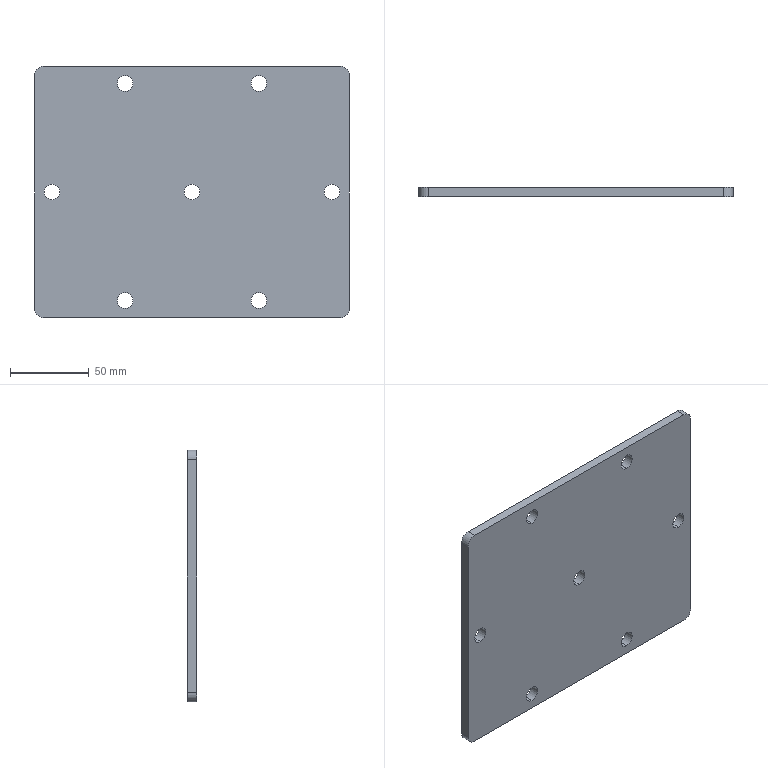Component | SolidWorks | UpperHousingAssembly-1_PeepHoleCover-1 | 1 solid | 24 faces | box 200 x 6 x 160 mm | volume 188516 mm3 | cylinder 18 | plane 6 | commonest cylinder face diameters 10 x14 12 x4
build123d program:
from build123d import *

# Parameters (mm, degrees)
SKETCH1_W           = 200
SKETCH1_H           = 160
BOSS_EXTRUDE1_DEPTH = 6
FILLET1_R           = 6
M10_TAPPED_HOLE1_D  = 10


with BuildPart() as part:
    # Sketch1 → Boss-Extrude1 (new body)
    with BuildSketch(Plane(origin=(0, 0, 0), x_dir=(1, 0, 0), z_dir=(0, 1, 0))):
        Rectangle(SKETCH1_W, SKETCH1_H)
    extrude(amount=BOSS_EXTRUDE1_DEPTH)

    # Fillet1
    fillet1_edges = [part.edges().sort_by_distance(p)[0] for p in [
        (100, 3, 80),
        (-100, 3, 80),
        (-100, 3, -80),
        (100, 3, -80),
    ]]
    fillet(fillet1_edges, radius=FILLET1_R)

    # M10 Tapped Hole1 (through all)
    with Locations(Plane(origin=(0, 6, 0), x_dir=(1, 0, 0), z_dir=(0, 1, 0))):
        with Locations((0, 0), (42.5, 69), (-42.5, 69), (-89, 0), (89, 0), (42.5, -69), (-42.5, -69)):
            Hole(M10_TAPPED_HOLE1_D / 2)


solid = part.part

# Placed as in the assembly
solid = solid.moved(Location((895.83, 1541.591, 1632.217), (0, 0, 0)))
STEP:
#1=COLOUR_RGB('',0.7922,0.8196,0.9333);
#2=FILL_AREA_STYLE_COLOUR('',#1);
#3=FILL_AREA_STYLE('',(#2));
#4=SURFACE_STYLE_FILL_AREA(#3);
#5=SURFACE_SIDE_STYLE('',(#4));
#6=SURFACE_STYLE_USAGE(.BOTH.,#5);
#7=PRESENTATION_STYLE_ASSIGNMENT((#6));
#8=CARTESIAN_POINT('',(35.269,60.693,64.064));
#9=VERTEX_POINT('',#8);
#10=CARTESIAN_POINT('',(35.269,60.693,64.457));
#11=VERTEX_POINT('',#10);
#12=CARTESIAN_POINT('',(35.269,60.693,64.26));
#13=DIRECTION('',(0.,1.,0.));
#14=DIRECTION('',(0.,0.,1.));
#15=AXIS2_PLACEMENT_3D('',#12,#13,#14);
#16=CIRCLE('',#15,0.1969);
#17=EDGE_CURVE('',#9,#11,#16,.T.);
#18=ORIENTED_EDGE('',*,*,#17,.F.);
#19=CARTESIAN_POINT('',(35.269,60.929,64.064));
#20=VERTEX_POINT('',#19);
#21=CARTESIAN_POINT('',(35.269,60.929,64.064));
#22=DIRECTION('',(0.,1.,0.));
#23=VECTOR('',#22,39.37);
#24=LINE('',#21,#23);
#25=EDGE_CURVE('',#9,#20,#24,.T.);
#26=ORIENTED_EDGE('',*,*,#25,.T.);
#27=CARTESIAN_POINT('',(35.269,60.929,64.457));
#28=VERTEX_POINT('',#27);
#29=CARTESIAN_POINT('',(35.269,60.929,64.26));
#30=DIRECTION('',(0.,1.,0.));
#31=DIRECTION('',(0.,0.,1.));
#32=AXIS2_PLACEMENT_3D('',#29,#30,#31);
#33=CIRCLE('',#32,0.1969);
#34=EDGE_CURVE('',#20,#28,#33,.T.);
#35=ORIENTED_EDGE('',*,*,#34,.T.);
#36=CARTESIAN_POINT('',(35.269,60.929,64.457));
#37=DIRECTION('',(0.,1.,0.));
#38=VECTOR('',#37,39.37);
#39=LINE('',#36,#38);
#40=EDGE_CURVE('',#11,#28,#39,.T.);
#41=ORIENTED_EDGE('',*,*,#40,.F.);
#42=EDGE_LOOP('',(#18,#26,#35,#41));
#43=FACE_OUTER_BOUND('',#42,.T.);
#44=CARTESIAN_POINT('',(35.269,60.929,64.26));
#45=DIRECTION('',(0.,1.,0.));
#46=DIRECTION('',(0.,0.,1.));
#47=AXIS2_PLACEMENT_3D('',#44,#45,#46);
#48=CYLINDRICAL_SURFACE('',#47,0.1969);
#49=ADVANCED_FACE('',(#43),#48,.F.);
#50=CARTESIAN_POINT('',(36.942,60.693,61.347));
#51=VERTEX_POINT('',#50);
#52=CARTESIAN_POINT('',(36.942,60.693,61.741));
#53=VERTEX_POINT('',#52);
#54=CARTESIAN_POINT('',(36.942,60.693,61.544));
#55=DIRECTION('',(0.,1.,0.));
#56=DIRECTION('',(0.,0.,1.));
#57=AXIS2_PLACEMENT_3D('',#54,#55,#56);
#58=CIRCLE('',#57,0.1969);
#59=EDGE_CURVE('',#51,#53,#58,.T.);
#60=ORIENTED_EDGE('',*,*,#59,.F.);
#61=CARTESIAN_POINT('',(36.942,60.929,61.347));
#62=VERTEX_POINT('',#61);
#63=CARTESIAN_POINT('',(36.942,60.929,61.347));
#64=DIRECTION('',(0.,1.,0.));
#65=VECTOR('',#64,39.37);
#66=LINE('',#63,#65);
#67=EDGE_CURVE('',#51,#62,#66,.T.);
#68=ORIENTED_EDGE('',*,*,#67,.T.);
#69=CARTESIAN_POINT('',(36.942,60.929,61.741));
#70=VERTEX_POINT('',#69);
#71=CARTESIAN_POINT('',(36.942,60.929,61.544));
#72=DIRECTION('',(0.,1.,0.));
#73=DIRECTION('',(0.,0.,1.));
#74=AXIS2_PLACEMENT_3D('',#71,#72,#73);
#75=CIRCLE('',#74,0.1969);
#76=EDGE_CURVE('',#62,#70,#75,.T.);
#77=ORIENTED_EDGE('',*,*,#76,.T.);
#78=CARTESIAN_POINT('',(36.942,60.929,61.741));
#79=DIRECTION('',(0.,1.,0.));
#80=VECTOR('',#79,39.37);
#81=LINE('',#78,#80);
#82=EDGE_CURVE('',#53,#70,#81,.T.);
#83=ORIENTED_EDGE('',*,*,#82,.F.);
#84=EDGE_LOOP('',(#60,#68,#77,#83));
#85=FACE_OUTER_BOUND('',#84,.T.);
#86=CARTESIAN_POINT('',(36.942,60.929,61.544));
#87=DIRECTION('',(0.,1.,0.));
#88=DIRECTION('',(0.,0.,1.));
#89=AXIS2_PLACEMENT_3D('',#86,#87,#88);
#90=CYLINDRICAL_SURFACE('',#89,0.1969);
#91=ADVANCED_FACE('',(#85),#90,.F.);
#92=CARTESIAN_POINT('',(33.596,60.693,61.347));
#93=VERTEX_POINT('',#92);
#94=CARTESIAN_POINT('',(33.596,60.693,61.741));
#95=VERTEX_POINT('',#94);
#96=CARTESIAN_POINT('',(33.596,60.693,61.544));
#97=DIRECTION('',(0.,1.,0.));
#98=DIRECTION('',(0.,0.,1.));
#99=AXIS2_PLACEMENT_3D('',#96,#97,#98);
#100=CIRCLE('',#99,0.1969);
#101=EDGE_CURVE('',#93,#95,#100,.T.);
#102=ORIENTED_EDGE('',*,*,#101,.F.);
#103=CARTESIAN_POINT('',(33.596,60.929,61.347));
#104=VERTEX_POINT('',#103);
#105=CARTESIAN_POINT('',(33.596,60.929,61.347));
#106=DIRECTION('',(0.,1.,0.));
#107=VECTOR('',#106,39.37);
#108=LINE('',#105,#107);
#109=EDGE_CURVE('',#93,#104,#108,.T.);
#110=ORIENTED_EDGE('',*,*,#109,.T.);
#111=CARTESIAN_POINT('',(33.596,60.929,61.741));
#112=VERTEX_POINT('',#111);
#113=CARTESIAN_POINT('',(33.596,60.929,61.544));
#114=DIRECTION('',(0.,1.,0.));
#115=DIRECTION('',(0.,0.,1.));
#116=AXIS2_PLACEMENT_3D('',#113,#114,#115);
#117=CIRCLE('',#116,0.1969);
#118=EDGE_CURVE('',#104,#112,#117,.T.);
#119=ORIENTED_EDGE('',*,*,#118,.T.);
#120=CARTESIAN_POINT('',(33.596,60.929,61.741));
#121=DIRECTION('',(0.,1.,0.));
#122=VECTOR('',#121,39.37);
#123=LINE('',#120,#122);
#124=EDGE_CURVE('',#95,#112,#123,.T.);
#125=ORIENTED_EDGE('',*,*,#124,.F.);
#126=EDGE_LOOP('',(#102,#110,#119,#125));
#127=FACE_OUTER_BOUND('',#126,.T.);
#128=CARTESIAN_POINT('',(33.596,60.929,61.544));
#129=DIRECTION('',(0.,1.,0.));
#130=DIRECTION('',(0.,0.,1.));
#131=AXIS2_PLACEMENT_3D('',#128,#129,#130);
#132=CYLINDRICAL_SURFACE('',#131,0.1969);
#133=ADVANCED_FACE('',(#127),#132,.F.);
#134=CARTESIAN_POINT('',(31.765,60.693,64.064));
#135=VERTEX_POINT('',#134);
#136=CARTESIAN_POINT('',(31.765,60.693,64.457));
#137=VERTEX_POINT('',#136);
#138=CARTESIAN_POINT('',(31.765,60.693,64.26));
#139=DIRECTION('',(0.,1.,0.));
#140=DIRECTION('',(0.,0.,1.));
#141=AXIS2_PLACEMENT_3D('',#138,#139,#140);
#142=CIRCLE('',#141,0.1969);
#143=EDGE_CURVE('',#135,#137,#142,.T.);
#144=ORIENTED_EDGE('',*,*,#143,.F.);
#145=CARTESIAN_POINT('',(31.765,60.929,64.064));
#146=VERTEX_POINT('',#145);
#147=CARTESIAN_POINT('',(31.765,60.929,64.064));
#148=DIRECTION('',(0.,1.,0.));
#149=VECTOR('',#148,39.37);
#150=LINE('',#147,#149);
#151=EDGE_CURVE('',#135,#146,#150,.T.);
#152=ORIENTED_EDGE('',*,*,#151,.T.);
#153=CARTESIAN_POINT('',(31.765,60.929,64.457));
#154=VERTEX_POINT('',#153);
#155=CARTESIAN_POINT('',(31.765,60.929,64.26));
#156=DIRECTION('',(0.,1.,0.));
#157=DIRECTION('',(0.,0.,1.));
#158=AXIS2_PLACEMENT_3D('',#155,#156,#157);
#159=CIRCLE('',#158,0.1969);
#160=EDGE_CURVE('',#146,#154,#159,.T.);
#161=ORIENTED_EDGE('',*,*,#160,.T.);
#162=CARTESIAN_POINT('',(31.765,60.929,64.457));
#163=DIRECTION('',(0.,1.,0.));
#164=VECTOR('',#163,39.37);
#165=LINE('',#162,#164);
#166=EDGE_CURVE('',#137,#154,#165,.T.);
#167=ORIENTED_EDGE('',*,*,#166,.F.);
#168=EDGE_LOOP('',(#144,#152,#161,#167));
#169=FACE_OUTER_BOUND('',#168,.T.);
#170=CARTESIAN_POINT('',(31.765,60.929,64.26));
#171=DIRECTION('',(0.,1.,0.));
#172=DIRECTION('',(0.,0.,1.));
#173=AXIS2_PLACEMENT_3D('',#170,#171,#172);
#174=CYLINDRICAL_SURFACE('',#173,0.1969);
#175=ADVANCED_FACE('',(#169),#174,.F.);
#176=CARTESIAN_POINT('',(38.773,60.693,64.064));
#177=VERTEX_POINT('',#176);
#178=CARTESIAN_POINT('',(38.773,60.693,64.457));
#179=VERTEX_POINT('',#178);
#180=CARTESIAN_POINT('',(38.773,60.693,64.26));
#181=DIRECTION('',(0.,1.,0.));
#182=DIRECTION('',(0.,0.,1.));
#183=AXIS2_PLACEMENT_3D('',#180,#181,#182);
#184=CIRCLE('',#183,0.1969);
#185=EDGE_CURVE('',#177,#179,#184,.T.);
#186=ORIENTED_EDGE('',*,*,#185,.F.);
#187=CARTESIAN_POINT('',(38.773,60.929,64.064));
#188=VERTEX_POINT('',#187);
#189=CARTESIAN_POINT('',(38.773,60.929,64.064));
#190=DIRECTION('',(0.,1.,0.));
#191=VECTOR('',#190,39.37);
#192=LINE('',#189,#191);
#193=EDGE_CURVE('',#177,#188,#192,.T.);
#194=ORIENTED_EDGE('',*,*,#193,.T.);
#195=CARTESIAN_POINT('',(38.773,60.929,64.457));
#196=VERTEX_POINT('',#195);
#197=CARTESIAN_POINT('',(38.773,60.929,64.26));
#198=DIRECTION('',(0.,1.,0.));
#199=DIRECTION('',(0.,0.,1.));
#200=AXIS2_PLACEMENT_3D('',#197,#198,#199);
#201=CIRCLE('',#200,0.1969);
#202=EDGE_CURVE('',#188,#196,#201,.T.);
#203=ORIENTED_EDGE('',*,*,#202,.T.);
#204=CARTESIAN_POINT('',(38.773,60.929,64.457));
#205=DIRECTION('',(0.,1.,0.));
#206=VECTOR('',#205,39.37);
#207=LINE('',#204,#206);
#208=EDGE_CURVE('',#179,#196,#207,.T.);
#209=ORIENTED_EDGE('',*,*,#208,.F.);
#210=EDGE_LOOP('',(#186,#194,#203,#209));
#211=FACE_OUTER_BOUND('',#210,.T.);
#212=CARTESIAN_POINT('',(38.773,60.929,64.26));
#213=DIRECTION('',(0.,1.,0.));
#214=DIRECTION('',(0.,0.,1.));
#215=AXIS2_PLACEMENT_3D('',#212,#213,#214);
#216=CYLINDRICAL_SURFACE('',#215,0.1969);
#217=ADVANCED_FACE('',(#211),#216,.F.);
#218=CARTESIAN_POINT('',(36.942,60.693,66.78));
#219=VERTEX_POINT('',#218);
#220=CARTESIAN_POINT('',(36.942,60.693,67.174));
#221=VERTEX_POINT('',#220);
#222=CARTESIAN_POINT('',(36.942,60.693,66.977));
#223=DIRECTION('',(0.,1.,0.));
#224=DIRECTION('',(0.,0.,1.));
#225=AXIS2_PLACEMENT_3D('',#222,#223,#224);
#226=CIRCLE('',#225,0.1969);
#227=EDGE_CURVE('',#219,#221,#226,.T.);
#228=ORIENTED_EDGE('',*,*,#227,.F.);
#229=CARTESIAN_POINT('',(36.942,60.929,66.78));
#230=VERTEX_POINT('',#229);
#231=CARTESIAN_POINT('',(36.942,60.929,66.78));
#232=DIRECTION('',(0.,1.,0.));
#233=VECTOR('',#232,39.37);
#234=LINE('',#231,#233);
#235=EDGE_CURVE('',#219,#230,#234,.T.);
#236=ORIENTED_EDGE('',*,*,#235,.T.);
#237=CARTESIAN_POINT('',(36.942,60.929,67.174));
#238=VERTEX_POINT('',#237);
#239=CARTESIAN_POINT('',(36.942,60.929,66.977));
#240=DIRECTION('',(0.,1.,0.));
#241=DIRECTION('',(0.,0.,1.));
#242=AXIS2_PLACEMENT_3D('',#239,#240,#241);
#243=CIRCLE('',#242,0.1969);
#244=EDGE_CURVE('',#230,#238,#243,.T.);
#245=ORIENTED_EDGE('',*,*,#244,.T.);
#246=CARTESIAN_POINT('',(36.942,60.929,67.174));
#247=DIRECTION('',(0.,1.,0.));
#248=VECTOR('',#247,39.37);
#249=LINE('',#246,#248);
#250=EDGE_CURVE('',#221,#238,#249,.T.);
#251=ORIENTED_EDGE('',*,*,#250,.F.);
#252=EDGE_LOOP('',(#228,#236,#245,#251));
#253=FACE_OUTER_BOUND('',#252,.T.);
#254=CARTESIAN_POINT('',(36.942,60.929,66.977));
#255=DIRECTION('',(0.,1.,0.));
#256=DIRECTION('',(0.,0.,1.));
#257=AXIS2_PLACEMENT_3D('',#254,#255,#256);
#258=CYLINDRICAL_SURFACE('',#257,0.1969);
#259=ADVANCED_FACE('',(#253),#258,.F.);
#260=CARTESIAN_POINT('',(33.596,60.693,66.78));
#261=VERTEX_POINT('',#260);
#262=CARTESIAN_POINT('',(33.596,60.693,67.174));
#263=VERTEX_POINT('',#262);
#264=CARTESIAN_POINT('',(33.596,60.693,66.977));
#265=DIRECTION('',(0.,1.,0.));
#266=DIRECTION('',(0.,0.,1.));
#267=AXIS2_PLACEMENT_3D('',#264,#265,#266);
#268=CIRCLE('',#267,0.1969);
#269=EDGE_CURVE('',#261,#263,#268,.T.);
#270=ORIENTED_EDGE('',*,*,#269,.F.);
#271=CARTESIAN_POINT('',(33.596,60.929,66.78));
#272=VERTEX_POINT('',#271);
#273=CARTESIAN_POINT('',(33.596,60.929,66.78));
#274=DIRECTION('',(0.,1.,0.));
#275=VECTOR('',#274,39.37);
#276=LINE('',#273,#275);
#277=EDGE_CURVE('',#261,#272,#276,.T.);
#278=ORIENTED_EDGE('',*,*,#277,.T.);
#279=CARTESIAN_POINT('',(33.596,60.929,67.174));
#280=VERTEX_POINT('',#279);
#281=CARTESIAN_POINT('',(33.596,60.929,66.977));
#282=DIRECTION('',(0.,1.,0.));
#283=DIRECTION('',(0.,0.,1.));
#284=AXIS2_PLACEMENT_3D('',#281,#282,#283);
#285=CIRCLE('',#284,0.1969);
#286=EDGE_CURVE('',#272,#280,#285,.T.);
#287=ORIENTED_EDGE('',*,*,#286,.T.);
#288=CARTESIAN_POINT('',(33.596,60.929,67.174));
#289=DIRECTION('',(0.,1.,0.));
#290=VECTOR('',#289,39.37);
#291=LINE('',#288,#290);
#292=EDGE_CURVE('',#263,#280,#291,.T.);
#293=ORIENTED_EDGE('',*,*,#292,.F.);
#294=EDGE_LOOP('',(#270,#278,#287,#293));
#295=FACE_OUTER_BOUND('',#294,.T.);
#296=CARTESIAN_POINT('',(33.596,60.929,66.977));
#297=DIRECTION('',(0.,1.,0.));
#298=DIRECTION('',(0.,0.,1.));
#299=AXIS2_PLACEMENT_3D('',#296,#297,#298);
#300=CYLINDRICAL_SURFACE('',#299,0.1969);
#301=ADVANCED_FACE('',(#295),#300,.F.);
#302=CARTESIAN_POINT('',(39.206,60.693,67.174));
#303=VERTEX_POINT('',#302);
#304=CARTESIAN_POINT('',(39.206,60.693,61.347));
#305=VERTEX_POINT('',#304);
#306=CARTESIAN_POINT('',(39.206,60.693,67.41));
#307=DIRECTION('',(0.,0.,-1.));
#308=VECTOR('',#307,39.37);
#309=LINE('',#306,#308);
#310=EDGE_CURVE('',#303,#305,#309,.T.);
#311=ORIENTED_EDGE('',*,*,#310,.T.);
#312=CARTESIAN_POINT('',(39.206,60.929,61.347));
#313=VERTEX_POINT('',#312);
#314=CARTESIAN_POINT('',(39.206,60.929,61.347));
#315=DIRECTION('',(0.,1.,0.));
#316=VECTOR('',#315,39.37);
#317=LINE('',#314,#316);
#318=EDGE_CURVE('',#305,#313,#317,.T.);
#319=ORIENTED_EDGE('',*,*,#318,.T.);
#320=CARTESIAN_POINT('',(39.206,60.929,67.174));
#321=VERTEX_POINT('',#320);
#322=CARTESIAN_POINT('',(39.206,60.929,67.41));
#323=DIRECTION('',(0.,0.,-1.));
#324=VECTOR('',#323,39.37);
#325=LINE('',#322,#324);
#326=EDGE_CURVE('',#321,#313,#325,.T.);
#327=ORIENTED_EDGE('',*,*,#326,.F.);
#328=CARTESIAN_POINT('',(39.206,60.929,67.174));
#329=DIRECTION('',(0.,-1.,0.));
#330=VECTOR('',#329,39.37);
#331=LINE('',#328,#330);
#332=EDGE_CURVE('',#321,#303,#331,.T.);
#333=ORIENTED_EDGE('',*,*,#332,.T.);
#334=EDGE_LOOP('',(#311,#319,#327,#333));
#335=FACE_OUTER_BOUND('',#334,.T.);
#336=CARTESIAN_POINT('',(39.206,60.929,67.41));
#337=DIRECTION('',(-1.,0.,0.));
#338=DIRECTION('',(0.,0.,1.));
#339=AXIS2_PLACEMENT_3D('',#336,#337,#338);
#340=PLANE('',#339);
#341=ADVANCED_FACE('',(#335),#340,.F.);
#342=CARTESIAN_POINT('',(38.97,60.693,61.111));
#343=VERTEX_POINT('',#342);
#344=CARTESIAN_POINT('',(31.568,60.693,61.111));
#345=VERTEX_POINT('',#344);
#346=CARTESIAN_POINT('',(31.332,60.693,61.111));
#347=DIRECTION('',(-1.,0.,0.));
#348=VECTOR('',#347,39.37);
#349=LINE('',#346,#348);
#350=EDGE_CURVE('',#343,#345,#349,.T.);
#351=ORIENTED_EDGE('',*,*,#350,.T.);
#352=CARTESIAN_POINT('',(31.568,60.929,61.111));
#353=VERTEX_POINT('',#352);
#354=CARTESIAN_POINT('',(31.568,60.929,61.111));
#355=DIRECTION('',(0.,1.,0.));
#356=VECTOR('',#355,39.37);
#357=LINE('',#354,#356);
#358=EDGE_CURVE('',#345,#353,#357,.T.);
#359=ORIENTED_EDGE('',*,*,#358,.T.);
#360=CARTESIAN_POINT('',(38.97,60.929,61.111));
#361=VERTEX_POINT('',#360);
#362=CARTESIAN_POINT('',(31.332,60.929,61.111));
#363=DIRECTION('',(-1.,0.,0.));
#364=VECTOR('',#363,39.37);
#365=LINE('',#362,#364);
#366=EDGE_CURVE('',#361,#353,#365,.T.);
#367=ORIENTED_EDGE('',*,*,#366,.F.);
#368=CARTESIAN_POINT('',(38.97,60.929,61.111));
#369=DIRECTION('',(0.,-1.,0.));
#370=VECTOR('',#369,39.37);
#371=LINE('',#368,#370);
#372=EDGE_CURVE('',#361,#343,#371,.T.);
#373=ORIENTED_EDGE('',*,*,#372,.T.);
#374=EDGE_LOOP('',(#351,#359,#367,#373));
#375=FACE_OUTER_BOUND('',#374,.T.);
#376=CARTESIAN_POINT('',(31.332,60.929,61.111));
#377=DIRECTION('',(0.,0.,1.));
#378=DIRECTION('',(1.,0.,0.));
#379=AXIS2_PLACEMENT_3D('',#376,#377,#378);
#380=PLANE('',#379);
#381=ADVANCED_FACE('',(#375),#380,.F.);
#382=CARTESIAN_POINT('',(31.332,60.929,61.347));
#383=VERTEX_POINT('',#382);
#384=CARTESIAN_POINT('',(31.332,60.929,67.174));
#385=VERTEX_POINT('',#384);
#386=CARTESIAN_POINT('',(31.332,60.929,67.41));
#387=DIRECTION('',(0.,0.,1.));
#388=VECTOR('',#387,39.37);
#389=LINE('',#386,#388);
#390=EDGE_CURVE('',#383,#385,#389,.T.);
#391=ORIENTED_EDGE('',*,*,#390,.F.);
#392=CARTESIAN_POINT('',(31.332,60.693,61.347));
#393=VERTEX_POINT('',#392);
#394=CARTESIAN_POINT('',(31.332,60.929,61.347));
#395=DIRECTION('',(0.,-1.,0.));
#396=VECTOR('',#395,39.37);
#397=LINE('',#394,#396);
#398=EDGE_CURVE('',#383,#393,#397,.T.);
#399=ORIENTED_EDGE('',*,*,#398,.T.);
#400=CARTESIAN_POINT('',(31.332,60.693,67.174));
#401=VERTEX_POINT('',#400);
#402=CARTESIAN_POINT('',(31.332,60.693,67.41));
#403=DIRECTION('',(0.,0.,1.));
#404=VECTOR('',#403,39.37);
#405=LINE('',#402,#404);
#406=EDGE_CURVE('',#393,#401,#405,.T.);
#407=ORIENTED_EDGE('',*,*,#406,.T.);
#408=CARTESIAN_POINT('',(31.332,60.929,67.174));
#409=DIRECTION('',(0.,1.,0.));
#410=VECTOR('',#409,39.37);
#411=LINE('',#408,#410);
#412=EDGE_CURVE('',#401,#385,#411,.T.);
#413=ORIENTED_EDGE('',*,*,#412,.T.);
#414=EDGE_LOOP('',(#391,#399,#407,#413));
#415=FACE_OUTER_BOUND('',#414,.T.);
#416=CARTESIAN_POINT('',(31.332,60.929,67.41));
#417=DIRECTION('',(1.,0.,0.));
#418=DIRECTION('',(0.,0.,-1.));
#419=AXIS2_PLACEMENT_3D('',#416,#417,#418);
#420=PLANE('',#419);
#421=ADVANCED_FACE('',(#415),#420,.F.);
#422=CARTESIAN_POINT('',(31.568,60.693,67.41));
#423=VERTEX_POINT('',#422);
#424=CARTESIAN_POINT('',(38.97,60.693,67.41));
#425=VERTEX_POINT('',#424);
#426=CARTESIAN_POINT('',(31.332,60.693,67.41));
#427=DIRECTION('',(1.,0.,0.));
#428=VECTOR('',#427,39.37);
#429=LINE('',#426,#428);
#430=EDGE_CURVE('',#423,#425,#429,.T.);
#431=ORIENTED_EDGE('',*,*,#430,.T.);
#432=CARTESIAN_POINT('',(38.97,60.929,67.41));
#433=VERTEX_POINT('',#432);
#434=CARTESIAN_POINT('',(38.97,60.929,67.41));
#435=DIRECTION('',(0.,1.,0.));
#436=VECTOR('',#435,39.37);
#437=LINE('',#434,#436);
#438=EDGE_CURVE('',#425,#433,#437,.T.);
#439=ORIENTED_EDGE('',*,*,#438,.T.);
#440=CARTESIAN_POINT('',(31.568,60.929,67.41));
#441=VERTEX_POINT('',#440);
#442=CARTESIAN_POINT('',(31.332,60.929,67.41));
#443=DIRECTION('',(1.,0.,0.));
#444=VECTOR('',#443,39.37);
#445=LINE('',#442,#444);
#446=EDGE_CURVE('',#441,#433,#445,.T.);
#447=ORIENTED_EDGE('',*,*,#446,.F.);
#448=CARTESIAN_POINT('',(31.568,60.929,67.41));
#449=DIRECTION('',(0.,-1.,0.));
#450=VECTOR('',#449,39.37);
#451=LINE('',#448,#450);
#452=EDGE_CURVE('',#441,#423,#451,.T.);
#453=ORIENTED_EDGE('',*,*,#452,.T.);
#454=EDGE_LOOP('',(#431,#439,#447,#453));
#455=FACE_OUTER_BOUND('',#454,.T.);
#456=CARTESIAN_POINT('',(31.332,60.929,67.41));
#457=DIRECTION('',(0.,0.,-1.));
#458=DIRECTION('',(-1.,0.,0.));
#459=AXIS2_PLACEMENT_3D('',#456,#457,#458);
#460=PLANE('',#459);
#461=ADVANCED_FACE('',(#455),#460,.F.);
#462=CARTESIAN_POINT('',(35.269,60.929,64.26));
#463=DIRECTION('',(0.,1.,0.));
#464=DIRECTION('',(0.,0.,1.));
#465=AXIS2_PLACEMENT_3D('',#462,#463,#464);
#466=CIRCLE('',#465,0.1969);
#467=EDGE_CURVE('',#28,#20,#466,.T.);
#468=ORIENTED_EDGE('',*,*,#467,.F.);
#469=ORIENTED_EDGE('',*,*,#34,.F.);
#470=EDGE_LOOP('',(#468,#469));
#471=FACE_BOUND('',#470,.T.);
#472=CARTESIAN_POINT('',(36.942,60.929,61.544));
#473=DIRECTION('',(0.,1.,0.));
#474=DIRECTION('',(0.,0.,1.));
#475=AXIS2_PLACEMENT_3D('',#472,#473,#474);
#476=CIRCLE('',#475,0.1969);
#477=EDGE_CURVE('',#70,#62,#476,.T.);
#478=ORIENTED_EDGE('',*,*,#477,.F.);
#479=ORIENTED_EDGE('',*,*,#76,.F.);
#480=EDGE_LOOP('',(#478,#479));
#481=FACE_BOUND('',#480,.T.);
#482=CARTESIAN_POINT('',(33.596,60.929,61.544));
#483=DIRECTION('',(0.,1.,0.));
#484=DIRECTION('',(0.,0.,1.));
#485=AXIS2_PLACEMENT_3D('',#482,#483,#484);
#486=CIRCLE('',#485,0.1969);
#487=EDGE_CURVE('',#112,#104,#486,.T.);
#488=ORIENTED_EDGE('',*,*,#487,.F.);
#489=ORIENTED_EDGE('',*,*,#118,.F.);
#490=EDGE_LOOP('',(#488,#489));
#491=FACE_BOUND('',#490,.T.);
#492=CARTESIAN_POINT('',(31.765,60.929,64.26));
#493=DIRECTION('',(0.,1.,0.));
#494=DIRECTION('',(0.,0.,1.));
#495=AXIS2_PLACEMENT_3D('',#492,#493,#494);
#496=CIRCLE('',#495,0.1969);
#497=EDGE_CURVE('',#154,#146,#496,.T.);
#498=ORIENTED_EDGE('',*,*,#497,.F.);
#499=ORIENTED_EDGE('',*,*,#160,.F.);
#500=EDGE_LOOP('',(#498,#499));
#501=FACE_BOUND('',#500,.T.);
#502=CARTESIAN_POINT('',(38.773,60.929,64.26));
#503=DIRECTION('',(0.,1.,0.));
#504=DIRECTION('',(0.,0.,1.));
#505=AXIS2_PLACEMENT_3D('',#502,#503,#504);
#506=CIRCLE('',#505,0.1969);
#507=EDGE_CURVE('',#196,#188,#506,.T.);
#508=ORIENTED_EDGE('',*,*,#507,.F.);
#509=ORIENTED_EDGE('',*,*,#202,.F.);
#510=EDGE_LOOP('',(#508,#509));
#511=FACE_BOUND('',#510,.T.);
#512=CARTESIAN_POINT('',(36.942,60.929,66.977));
#513=DIRECTION('',(0.,1.,0.));
#514=DIRECTION('',(0.,0.,1.));
#515=AXIS2_PLACEMENT_3D('',#512,#513,#514);
#516=CIRCLE('',#515,0.1969);
#517=EDGE_CURVE('',#238,#230,#516,.T.);
#518=ORIENTED_EDGE('',*,*,#517,.F.);
#519=ORIENTED_EDGE('',*,*,#244,.F.);
#520=EDGE_LOOP('',(#518,#519));
#521=FACE_BOUND('',#520,.T.);
#522=CARTESIAN_POINT('',(33.596,60.929,66.977));
#523=DIRECTION('',(0.,1.,0.));
#524=DIRECTION('',(0.,0.,1.));
#525=AXIS2_PLACEMENT_3D('',#522,#523,#524);
#526=CIRCLE('',#525,0.1969);
#527=EDGE_CURVE('',#280,#272,#526,.T.);
#528=ORIENTED_EDGE('',*,*,#527,.F.);
#529=ORIENTED_EDGE('',*,*,#286,.F.);
#530=EDGE_LOOP('',(#528,#529));
#531=FACE_BOUND('',#530,.T.);
#532=ORIENTED_EDGE('',*,*,#366,.T.);
#533=CARTESIAN_POINT('',(31.568,60.929,61.347));
#534=DIRECTION('',(0.,1.,0.));
#535=DIRECTION('',(0.,0.,-1.));
#536=AXIS2_PLACEMENT_3D('',#533,#534,#535);
#537=CIRCLE('',#536,0.2362);
#538=EDGE_CURVE('',#353,#383,#537,.T.);
#539=ORIENTED_EDGE('',*,*,#538,.T.);
#540=ORIENTED_EDGE('',*,*,#390,.T.);
#541=CARTESIAN_POINT('',(31.568,60.929,67.174));
#542=DIRECTION('',(0.,1.,0.));
#543=DIRECTION('',(0.,0.,-1.));
#544=AXIS2_PLACEMENT_3D('',#541,#542,#543);
#545=CIRCLE('',#544,0.2362);
#546=EDGE_CURVE('',#385,#441,#545,.T.);
#547=ORIENTED_EDGE('',*,*,#546,.T.);
#548=ORIENTED_EDGE('',*,*,#446,.T.);
#549=CARTESIAN_POINT('',(38.97,60.929,67.174));
#550=DIRECTION('',(0.,1.,0.));
#551=DIRECTION('',(0.,0.,-1.));
#552=AXIS2_PLACEMENT_3D('',#549,#550,#551);
#553=CIRCLE('',#552,0.2362);
#554=EDGE_CURVE('',#433,#321,#553,.T.);
#555=ORIENTED_EDGE('',*,*,#554,.T.);
#556=ORIENTED_EDGE('',*,*,#326,.T.);
#557=CARTESIAN_POINT('',(38.97,60.929,61.347));
#558=DIRECTION('',(0.,1.,0.));
#559=DIRECTION('',(0.,0.,-1.));
#560=AXIS2_PLACEMENT_3D('',#557,#558,#559);
#561=CIRCLE('',#560,0.2362);
#562=EDGE_CURVE('',#313,#361,#561,.T.);
#563=ORIENTED_EDGE('',*,*,#562,.T.);
#564=EDGE_LOOP('',(#532,#539,#540,#547,#548,#555,#556,#563));
#565=FACE_OUTER_BOUND('',#564,.T.);
#566=CARTESIAN_POINT('',(35.269,60.929,64.26));
#567=DIRECTION('',(0.,-1.,0.));
#568=DIRECTION('',(0.,0.,-1.));
#569=AXIS2_PLACEMENT_3D('',#566,#567,#568);
#570=PLANE('',#569);
#571=ADVANCED_FACE('',(#471,#481,#491,#501,#511,#521,#531,#565),#570,.F.);
#572=CARTESIAN_POINT('',(35.269,60.693,64.26));
#573=DIRECTION('',(0.,1.,0.));
#574=DIRECTION('',(0.,0.,1.));
#575=AXIS2_PLACEMENT_3D('',#572,#573,#574);
#576=CIRCLE('',#575,0.1969);
#577=EDGE_CURVE('',#11,#9,#576,.T.);
#578=ORIENTED_EDGE('',*,*,#577,.T.);
#579=ORIENTED_EDGE('',*,*,#17,.T.);
#580=EDGE_LOOP('',(#578,#579));
#581=FACE_BOUND('',#580,.T.);
#582=CARTESIAN_POINT('',(36.942,60.693,61.544));
#583=DIRECTION('',(0.,1.,0.));
#584=DIRECTION('',(0.,0.,1.));
#585=AXIS2_PLACEMENT_3D('',#582,#583,#584);
#586=CIRCLE('',#585,0.1969);
#587=EDGE_CURVE('',#53,#51,#586,.T.);
#588=ORIENTED_EDGE('',*,*,#587,.T.);
#589=ORIENTED_EDGE('',*,*,#59,.T.);
#590=EDGE_LOOP('',(#588,#589));
#591=FACE_BOUND('',#590,.T.);
#592=CARTESIAN_POINT('',(33.596,60.693,61.544));
#593=DIRECTION('',(0.,1.,0.));
#594=DIRECTION('',(0.,0.,1.));
#595=AXIS2_PLACEMENT_3D('',#592,#593,#594);
#596=CIRCLE('',#595,0.1969);
#597=EDGE_CURVE('',#95,#93,#596,.T.);
#598=ORIENTED_EDGE('',*,*,#597,.T.);
#599=ORIENTED_EDGE('',*,*,#101,.T.);
#600=EDGE_LOOP('',(#598,#599));
#601=FACE_BOUND('',#600,.T.);
#602=CARTESIAN_POINT('',(31.765,60.693,64.26));
#603=DIRECTION('',(0.,1.,0.));
#604=DIRECTION('',(0.,0.,1.));
#605=AXIS2_PLACEMENT_3D('',#602,#603,#604);
#606=CIRCLE('',#605,0.1969);
#607=EDGE_CURVE('',#137,#135,#606,.T.);
#608=ORIENTED_EDGE('',*,*,#607,.T.);
#609=ORIENTED_EDGE('',*,*,#143,.T.);
#610=EDGE_LOOP('',(#608,#609));
#611=FACE_BOUND('',#610,.T.);
#612=CARTESIAN_POINT('',(38.773,60.693,64.26));
#613=DIRECTION('',(0.,1.,0.));
#614=DIRECTION('',(0.,0.,1.));
#615=AXIS2_PLACEMENT_3D('',#612,#613,#614);
#616=CIRCLE('',#615,0.1969);
#617=EDGE_CURVE('',#179,#177,#616,.T.);
#618=ORIENTED_EDGE('',*,*,#617,.T.);
#619=ORIENTED_EDGE('',*,*,#185,.T.);
#620=EDGE_LOOP('',(#618,#619));
#621=FACE_BOUND('',#620,.T.);
#622=CARTESIAN_POINT('',(36.942,60.693,66.977));
#623=DIRECTION('',(0.,1.,0.));
#624=DIRECTION('',(0.,0.,1.));
#625=AXIS2_PLACEMENT_3D('',#622,#623,#624);
#626=CIRCLE('',#625,0.1969);
#627=EDGE_CURVE('',#221,#219,#626,.T.);
#628=ORIENTED_EDGE('',*,*,#627,.T.);
#629=ORIENTED_EDGE('',*,*,#227,.T.);
#630=EDGE_LOOP('',(#628,#629));
#631=FACE_BOUND('',#630,.T.);
#632=CARTESIAN_POINT('',(33.596,60.693,66.977));
#633=DIRECTION('',(0.,1.,0.));
#634=DIRECTION('',(0.,0.,1.));
#635=AXIS2_PLACEMENT_3D('',#632,#633,#634);
#636=CIRCLE('',#635,0.1969);
#637=EDGE_CURVE('',#263,#261,#636,.T.);
#638=ORIENTED_EDGE('',*,*,#637,.T.);
#639=ORIENTED_EDGE('',*,*,#269,.T.);
#640=EDGE_LOOP('',(#638,#639));
#641=FACE_BOUND('',#640,.T.);
#642=ORIENTED_EDGE('',*,*,#406,.F.);
#643=CARTESIAN_POINT('',(31.568,60.693,61.347));
#644=DIRECTION('',(0.,-1.,0.));
#645=DIRECTION('',(0.,0.,-1.));
#646=AXIS2_PLACEMENT_3D('',#643,#644,#645);
#647=CIRCLE('',#646,0.2362);
#648=EDGE_CURVE('',#393,#345,#647,.T.);
#649=ORIENTED_EDGE('',*,*,#648,.T.);
#650=ORIENTED_EDGE('',*,*,#350,.F.);
#651=CARTESIAN_POINT('',(38.97,60.693,61.347));
#652=DIRECTION('',(0.,-1.,0.));
#653=DIRECTION('',(0.,0.,-1.));
#654=AXIS2_PLACEMENT_3D('',#651,#652,#653);
#655=CIRCLE('',#654,0.2362);
#656=EDGE_CURVE('',#343,#305,#655,.T.);
#657=ORIENTED_EDGE('',*,*,#656,.T.);
#658=ORIENTED_EDGE('',*,*,#310,.F.);
#659=CARTESIAN_POINT('',(38.97,60.693,67.174));
#660=DIRECTION('',(0.,-1.,0.));
#661=DIRECTION('',(0.,0.,-1.));
#662=AXIS2_PLACEMENT_3D('',#659,#660,#661);
#663=CIRCLE('',#662,0.2362);
#664=EDGE_CURVE('',#303,#425,#663,.T.);
#665=ORIENTED_EDGE('',*,*,#664,.T.);
#666=ORIENTED_EDGE('',*,*,#430,.F.);
#667=CARTESIAN_POINT('',(31.568,60.693,67.174));
#668=DIRECTION('',(0.,-1.,0.));
#669=DIRECTION('',(0.,0.,-1.));
#670=AXIS2_PLACEMENT_3D('',#667,#668,#669);
#671=CIRCLE('',#670,0.2362);
#672=EDGE_CURVE('',#423,#401,#671,.T.);
#673=ORIENTED_EDGE('',*,*,#672,.T.);
#674=EDGE_LOOP('',(#642,#649,#650,#657,#658,#665,#666,#673));
#675=FACE_OUTER_BOUND('',#674,.T.);
#676=CARTESIAN_POINT('',(35.269,60.693,64.26));
#677=DIRECTION('',(0.,-1.,0.));
#678=DIRECTION('',(0.,0.,-1.));
#679=AXIS2_PLACEMENT_3D('',#676,#677,#678);
#680=PLANE('',#679);
#681=ADVANCED_FACE('',(#581,#591,#601,#611,#621,#631,#641,#675),#680,.T.);
#682=ORIENTED_EDGE('',*,*,#538,.F.);
#683=ORIENTED_EDGE('',*,*,#358,.F.);
#684=ORIENTED_EDGE('',*,*,#648,.F.);
#685=ORIENTED_EDGE('',*,*,#398,.F.);
#686=EDGE_LOOP('',(#682,#683,#684,#685));
#687=FACE_OUTER_BOUND('',#686,.T.);
#688=CARTESIAN_POINT('',(31.568,60.929,61.347));
#689=DIRECTION('',(0.,-1.,0.));
#690=DIRECTION('',(0.,0.,-1.));
#691=AXIS2_PLACEMENT_3D('',#688,#689,#690);
#692=CYLINDRICAL_SURFACE('',#691,0.2362);
#693=ADVANCED_FACE('',(#687),#692,.T.);
#694=ORIENTED_EDGE('',*,*,#562,.F.);
#695=ORIENTED_EDGE('',*,*,#318,.F.);
#696=ORIENTED_EDGE('',*,*,#656,.F.);
#697=ORIENTED_EDGE('',*,*,#372,.F.);
#698=EDGE_LOOP('',(#694,#695,#696,#697));
#699=FACE_OUTER_BOUND('',#698,.T.);
#700=CARTESIAN_POINT('',(38.97,60.929,61.347));
#701=DIRECTION('',(0.,-1.,0.));
#702=DIRECTION('',(0.,0.,-1.));
#703=AXIS2_PLACEMENT_3D('',#700,#701,#702);
#704=CYLINDRICAL_SURFACE('',#703,0.2362);
#705=ADVANCED_FACE('',(#699),#704,.T.);
#706=ORIENTED_EDGE('',*,*,#554,.F.);
#707=ORIENTED_EDGE('',*,*,#438,.F.);
#708=ORIENTED_EDGE('',*,*,#664,.F.);
#709=ORIENTED_EDGE('',*,*,#332,.F.);
#710=EDGE_LOOP('',(#706,#707,#708,#709));
#711=FACE_OUTER_BOUND('',#710,.T.);
#712=CARTESIAN_POINT('',(38.97,60.929,67.174));
#713=DIRECTION('',(0.,-1.,0.));
#714=DIRECTION('',(0.,0.,-1.));
#715=AXIS2_PLACEMENT_3D('',#712,#713,#714);
#716=CYLINDRICAL_SURFACE('',#715,0.2362);
#717=ADVANCED_FACE('',(#711),#716,.T.);
#718=ORIENTED_EDGE('',*,*,#546,.F.);
#719=ORIENTED_EDGE('',*,*,#412,.F.);
#720=ORIENTED_EDGE('',*,*,#672,.F.);
#721=ORIENTED_EDGE('',*,*,#452,.F.);
#722=EDGE_LOOP('',(#718,#719,#720,#721));
#723=FACE_OUTER_BOUND('',#722,.T.);
#724=CARTESIAN_POINT('',(31.568,60.929,67.174));
#725=DIRECTION('',(0.,-1.,0.));
#726=DIRECTION('',(0.,0.,-1.));
#727=AXIS2_PLACEMENT_3D('',#724,#725,#726);
#728=CYLINDRICAL_SURFACE('',#727,0.2362);
#729=ADVANCED_FACE('',(#723),#728,.T.);
#730=ORIENTED_EDGE('',*,*,#277,.F.);
#731=ORIENTED_EDGE('',*,*,#637,.F.);
#732=ORIENTED_EDGE('',*,*,#292,.T.);
#733=ORIENTED_EDGE('',*,*,#527,.T.);
#734=EDGE_LOOP('',(#730,#731,#732,#733));
#735=FACE_OUTER_BOUND('',#734,.T.);
#736=CARTESIAN_POINT('',(33.596,60.929,66.977));
#737=DIRECTION('',(0.,1.,0.));
#738=DIRECTION('',(0.,0.,1.));
#739=AXIS2_PLACEMENT_3D('',#736,#737,#738);
#740=CYLINDRICAL_SURFACE('',#739,0.1969);
#741=ADVANCED_FACE('',(#735),#740,.F.);
#742=ORIENTED_EDGE('',*,*,#235,.F.);
#743=ORIENTED_EDGE('',*,*,#627,.F.);
#744=ORIENTED_EDGE('',*,*,#250,.T.);
#745=ORIENTED_EDGE('',*,*,#517,.T.);
#746=EDGE_LOOP('',(#742,#743,#744,#745));
#747=FACE_OUTER_BOUND('',#746,.T.);
#748=CARTESIAN_POINT('',(36.942,60.929,66.977));
#749=DIRECTION('',(0.,1.,0.));
#750=DIRECTION('',(0.,0.,1.));
#751=AXIS2_PLACEMENT_3D('',#748,#749,#750);
#752=CYLINDRICAL_SURFACE('',#751,0.1969);
#753=ADVANCED_FACE('',(#747),#752,.F.);
#754=ORIENTED_EDGE('',*,*,#193,.F.);
#755=ORIENTED_EDGE('',*,*,#617,.F.);
#756=ORIENTED_EDGE('',*,*,#208,.T.);
#757=ORIENTED_EDGE('',*,*,#507,.T.);
#758=EDGE_LOOP('',(#754,#755,#756,#757));
#759=FACE_OUTER_BOUND('',#758,.T.);
#760=CARTESIAN_POINT('',(38.773,60.929,64.26));
#761=DIRECTION('',(0.,1.,0.));
#762=DIRECTION('',(0.,0.,1.));
#763=AXIS2_PLACEMENT_3D('',#760,#761,#762);
#764=CYLINDRICAL_SURFACE('',#763,0.1969);
#765=ADVANCED_FACE('',(#759),#764,.F.);
#766=ORIENTED_EDGE('',*,*,#151,.F.);
#767=ORIENTED_EDGE('',*,*,#607,.F.);
#768=ORIENTED_EDGE('',*,*,#166,.T.);
#769=ORIENTED_EDGE('',*,*,#497,.T.);
#770=EDGE_LOOP('',(#766,#767,#768,#769));
#771=FACE_OUTER_BOUND('',#770,.T.);
#772=CARTESIAN_POINT('',(31.765,60.929,64.26));
#773=DIRECTION('',(0.,1.,0.));
#774=DIRECTION('',(0.,0.,1.));
#775=AXIS2_PLACEMENT_3D('',#772,#773,#774);
#776=CYLINDRICAL_SURFACE('',#775,0.1969);
#777=ADVANCED_FACE('',(#771),#776,.F.);
#778=ORIENTED_EDGE('',*,*,#109,.F.);
#779=ORIENTED_EDGE('',*,*,#597,.F.);
#780=ORIENTED_EDGE('',*,*,#124,.T.);
#781=ORIENTED_EDGE('',*,*,#487,.T.);
#782=EDGE_LOOP('',(#778,#779,#780,#781));
#783=FACE_OUTER_BOUND('',#782,.T.);
#784=CARTESIAN_POINT('',(33.596,60.929,61.544));
#785=DIRECTION('',(0.,1.,0.));
#786=DIRECTION('',(0.,0.,1.));
#787=AXIS2_PLACEMENT_3D('',#784,#785,#786);
#788=CYLINDRICAL_SURFACE('',#787,0.1969);
#789=ADVANCED_FACE('',(#783),#788,.F.);
#790=ORIENTED_EDGE('',*,*,#67,.F.);
#791=ORIENTED_EDGE('',*,*,#587,.F.);
#792=ORIENTED_EDGE('',*,*,#82,.T.);
#793=ORIENTED_EDGE('',*,*,#477,.T.);
#794=EDGE_LOOP('',(#790,#791,#792,#793));
#795=FACE_OUTER_BOUND('',#794,.T.);
#796=CARTESIAN_POINT('',(36.942,60.929,61.544));
#797=DIRECTION('',(0.,1.,0.));
#798=DIRECTION('',(0.,0.,1.));
#799=AXIS2_PLACEMENT_3D('',#796,#797,#798);
#800=CYLINDRICAL_SURFACE('',#799,0.1969);
#801=ADVANCED_FACE('',(#795),#800,.F.);
#802=ORIENTED_EDGE('',*,*,#25,.F.);
#803=ORIENTED_EDGE('',*,*,#577,.F.);
#804=ORIENTED_EDGE('',*,*,#40,.T.);
#805=ORIENTED_EDGE('',*,*,#467,.T.);
#806=EDGE_LOOP('',(#802,#803,#804,#805));
#807=FACE_OUTER_BOUND('',#806,.T.);
#808=CARTESIAN_POINT('',(35.269,60.929,64.26));
#809=DIRECTION('',(0.,1.,0.));
#810=DIRECTION('',(0.,0.,1.));
#811=AXIS2_PLACEMENT_3D('',#808,#809,#810);
#812=CYLINDRICAL_SURFACE('',#811,0.1969);
#813=ADVANCED_FACE('',(#807),#812,.F.);
#814=CLOSED_SHELL('',(#49,#91,#133,#175,#217,#259,#301,#341,#381,#421,#461,#571,#681,#693,#705,#717,#729,#741,#753,#765,#777,#789,#801,#813));
#815=MANIFOLD_SOLID_BREP('',#814);
#816=STYLED_ITEM('',(#7),#815);
#817=(LENGTH_UNIT()NAMED_UNIT(*)SI_UNIT($,.METRE.));
#818=LENGTH_MEASURE_WITH_UNIT(LENGTH_MEASURE(0.0254),#817);
#819=DIMENSIONAL_EXPONENTS(1.,0.,0.,0.,0.,0.,0.);
#820=(CONVERSION_BASED_UNIT('',#818)LENGTH_UNIT()NAMED_UNIT(#819));
#821=UNCERTAINTY_MEASURE_WITH_UNIT(LENGTH_MEASURE(0.00001),#820,'','');
#822=(NAMED_UNIT(*)PLANE_ANGLE_UNIT()SI_UNIT($,.RADIAN.));
#823=(NAMED_UNIT(*)SI_UNIT($,.STERADIAN.)SOLID_ANGLE_UNIT());
#824=(GEOMETRIC_REPRESENTATION_CONTEXT(3)GLOBAL_UNCERTAINTY_ASSIGNED_CONTEXT((#821))GLOBAL_UNIT_ASSIGNED_CONTEXT((#820,#822,#823))REPRESENTATION_CONTEXT('',''));
#825=MECHANICAL_DESIGN_GEOMETRIC_PRESENTATION_REPRESENTATION('',(#816),#824);
#826=PRESENTATION_LAYER_ASSIGNMENT('','',(#816));
#827=CARTESIAN_POINT('',(0.,0.,0.));
#828=DIRECTION('',(0.,0.,1.));
#829=DIRECTION('',(1.,0.,0.));
#830=AXIS2_PLACEMENT_3D('',#827,#828,#829);
#831=(LENGTH_UNIT()NAMED_UNIT(*)SI_UNIT($,.METRE.));
#832=LENGTH_MEASURE_WITH_UNIT(LENGTH_MEASURE(0.0254),#831);
#833=DIMENSIONAL_EXPONENTS(1.,0.,0.,0.,0.,0.,0.);
#834=(CONVERSION_BASED_UNIT('',#832)LENGTH_UNIT()NAMED_UNIT(#833));
#835=UNCERTAINTY_MEASURE_WITH_UNIT(LENGTH_MEASURE(0.00001),#834,'','');
#836=(NAMED_UNIT(*)PLANE_ANGLE_UNIT()SI_UNIT($,.RADIAN.));
#837=(NAMED_UNIT(*)SI_UNIT($,.STERADIAN.)SOLID_ANGLE_UNIT());
#838=(GEOMETRIC_REPRESENTATION_CONTEXT(3)GLOBAL_UNCERTAINTY_ASSIGNED_CONTEXT((#835))GLOBAL_UNIT_ASSIGNED_CONTEXT((#834,#836,#837))REPRESENTATION_CONTEXT('',''));
#839=ADVANCED_BREP_SHAPE_REPRESENTATION('',(#815,#830),#838);